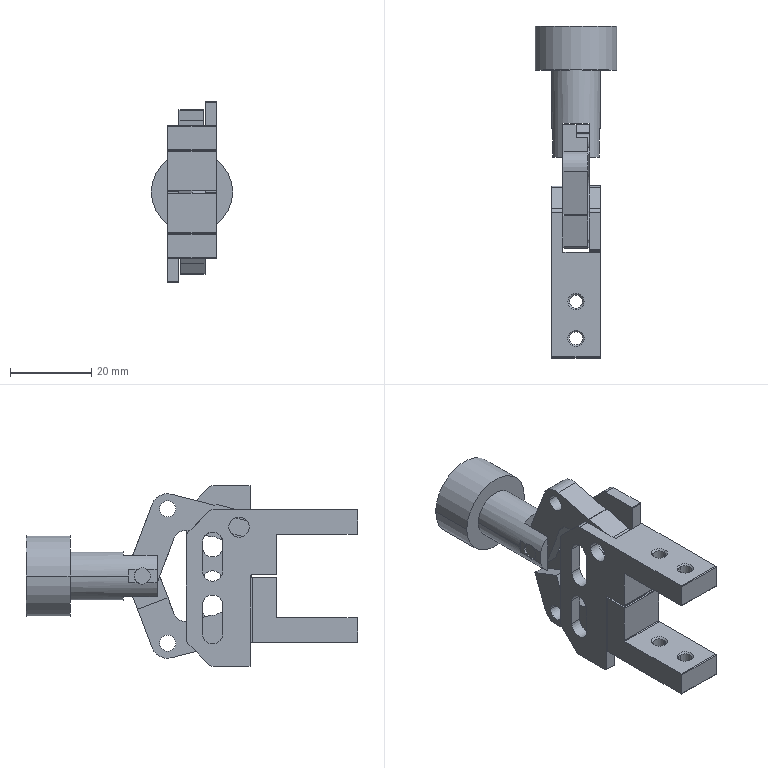Component | SolidWorks | CCDJSHFP20(NC)+(CS1-G-2)-1_CCDJSHFP20_finger(0)-1 | 1 solid | 194 faces | box 20 x 81.5 x 44.3 mm | volume 15573 mm3 | plane 107 | cylinder 71 | cone 16 | commonest cylinder face diameters 4 x16 5 x12 0.4 x12 3.242 x8 3 x8 1 x5 4.2 x2 20 x2
build123d program:
from build123d import *

# Parameters (mm, degrees)
CUT_EXTRUDE1_2_DEPTH      = 6
CUT_EXTRUDE1_2_DEPTH_BACK = 6
CUT_EXTRUDE2_DEPTH        = 6
CUT_EXTRUDE2_DEPTH_BACK   = 6
SKETCH3_R                 = 2
SKETCH4_R                 = 2
BOSS_EXTRUDE1_DEPTH       = 3.2
SKETCH5_R                 = 2
BOSS_EXTRUDE2_DEPTH       = 6.1
SKETCH6_R                 = 2
BOSS_EXTRUDE3_DEPTH       = 3.2
SKETCH7_R                 = 2
BOSS_EXTRUDE4_DEPTH       = 6.1
SKETCH8_R                 = 2.5
BOSS_EXTRUDE5_DEPTH       = 2.8
BOSS_EXTRUDE6_START       = 11.7
BOSS_EXTRUDE6_DEPTH       = 11.7
SKETCH10_R                = 2.5
BOSS_EXTRUDE7_DEPTH       = 2.8
BOSS_EXTRUDE8_DEPTH       = 12
BOSS_EXTRUDE9_DEPTH       = 5.35
BOSS_EXTRUDE9_DEPTH_BACK  = 5.35
SKETCH12_R                = 2.1
CUT_EXTRUDE1_DEPTH        = 66.663
CUT_EXTRUDE1_DEPTH_BACK   = 66.663
SKETCH1_R                 = 2


with BuildPart() as part:
    # Sketch1_2 → Revolve1 (revolve)
    with BuildSketch(Plane.XY, mode=Mode.PRIVATE) as revolve1_sk:
        Polygon((28.8, 0), (28.8, 6), (50.2, 6), (50.2, 10), (61, 10), (61, 0), align=None)
    revolve(revolve1_sk.sketch.rotate(Axis((61, 0, 0), (-1, 0, 0)), 270), axis=Axis((61, 0, 0), (-1, 0, 0)))

    # Sketch2 → Cut-Extrude1_2 (cut, two sides: drawn at the far end of the back side and taken through both)
    with BuildSketch(Plane(origin=(0, 0, 0), x_dir=(1, 0, 0), z_dir=(0, 1, 0)).offset(-CUT_EXTRUDE1_2_DEPTH_BACK)):
        Polygon((26.8, -6), (35.8, -6), (35.8, -5.75), (28.8, -5.75), (28.8, -3.2), (37.1, -3.2), (37.1, 3.2), (28.8, 3.2), (28.8, 5.75), (35.8, 5.75), (35.8, 6), (26.8, 6), align=None)
    extrude(amount=CUT_EXTRUDE1_2_DEPTH + CUT_EXTRUDE1_2_DEPTH_BACK, mode=Mode.SUBTRACT)

    # Sketch3 → Cut-Extrude2 (cut, two sides: drawn at the far end of the back side and taken through both)
    with BuildSketch(Plane.XY.offset(-CUT_EXTRUDE2_DEPTH_BACK)):
        with Locations(Location((32.45, 0, 0), (0, 0, 58.977))):
            Circle(SKETCH3_R)
    extrude(amount=CUT_EXTRUDE2_DEPTH + CUT_EXTRUDE2_DEPTH_BACK, mode=Mode.SUBTRACT)

    # Sketch4 → Boss-Extrude1 (add)
    with BuildSketch(Plane.XY.offset(-3.2)):
        with BuildLine():
            Line((20.984, 18.979), (29.329, -3.053))
            Line((29.329, -3.053), (31.2, -2.345))
            Line((31.2, -2.345), (29.96, 0.9281))
            ThreePointArc((29.96, 0.9281), (31.122, 3.507), (33.7, 2.345))
            Line((33.7, 2.345), (34.94, -0.9281))
            Line((34.94, -0.9281), (36.811, -0.2196))
            Line((36.811, -0.2196), (30.048, 17.635))
            ThreePointArc((30.048, 17.635), (28.149, 19.768), (25.311, 20.092))
            Line((25.311, 20.092), (20.984, 18.979))
        make_face()
        with Locations((26.2, 16.5)):
            Circle(SKETCH4_R, mode=Mode.SUBTRACT)
    extrude(amount=BOSS_EXTRUDE1_DEPTH)

    # Sketch5 → Boss-Extrude2 (add)
    with BuildSketch(Plane.XY.offset(-3.2)):
        with BuildLine():
            Line((6.434, 15.031), (6.807, 13.578))
            Line((6.807, 13.578), (9.229, 14.201))
            ThreePointArc((9.229, 14.201), (11.664, 12.762), (10.225, 10.327))
            Line((10.225, 10.327), (7.803, 9.704))
            Line((7.803, 9.704), (8.177, 8.252))
            ThreePointArc((8.177, 8.252), (8.407, 7.946), (8.786, 7.892))
            Line((8.786, 7.892), (21.127, 11.065))
            ThreePointArc((21.127, 11.065), (23.255, 10.823), (24.679, 9.223))
            Line((24.679, 9.223), (26.141, 5.363))
            Line((26.141, 5.363), (33.622, 8.197))
            Line((33.622, 8.197), (30.048, 17.635))
            ThreePointArc((30.048, 17.635), (28.149, 19.768), (25.311, 20.092))
            Line((25.311, 20.092), (14.713, 17.367))
            Line((14.713, 17.367), (14.348, 17.582))
            Line((14.348, 17.582), (6.793, 15.64))
            ThreePointArc((6.793, 15.64), (6.488, 15.41), (6.434, 15.031))
        make_face()
        with Locations((26.2, 16.5)):
            Circle(SKETCH5_R, mode=Mode.SUBTRACT)
    extrude(amount=BOSS_EXTRUDE2_DEPTH)

    # Sketch6 → Boss-Extrude3 (add)
    with BuildSketch(Plane.XY.offset(3.2)):
        with BuildLine():
            Line((20.984, -18.979), (25.311, -20.092))
            ThreePointArc((25.311, -20.092), (28.149, -19.768), (30.048, -17.635))
            Line((30.048, -17.635), (36.811, 0.2196))
            Line((36.811, 0.2196), (34.94, 0.9281))
            Line((34.94, 0.9281), (33.7, -2.345))
            ThreePointArc((33.7, -2.345), (31.122, -3.507), (29.96, -0.9281))
            Line((29.96, -0.9281), (31.2, 2.345))
            Line((31.2, 2.345), (29.329, 3.053))
            Line((29.329, 3.053), (20.984, -18.979))
        make_face()
        with Locations((26.2, -16.5)):
            Circle(SKETCH6_R, mode=Mode.SUBTRACT)
    extrude(amount=-BOSS_EXTRUDE3_DEPTH)

    # Sketch7 → Boss-Extrude4 (add)
    with BuildSketch(Plane.XY.offset(3.2)):
        with BuildLine():
            Line((6.793, -15.64), (14.348, -17.582))
            Line((14.348, -17.582), (14.713, -17.367))
            Line((14.713, -17.367), (25.311, -20.092))
            ThreePointArc((25.311, -20.092), (28.149, -19.768), (30.048, -17.635))
            Line((30.048, -17.635), (33.622, -8.197))
            Line((33.622, -8.197), (26.141, -5.363))
            Line((26.141, -5.363), (24.679, -9.223))
            ThreePointArc((24.679, -9.223), (23.255, -10.823), (21.127, -11.065))
            Line((21.127, -11.065), (8.786, -7.892))
            ThreePointArc((8.786, -7.892), (8.407, -7.946), (8.177, -8.252))
            Line((8.177, -8.252), (7.803, -9.704))
            Line((7.803, -9.704), (10.225, -10.327))
            ThreePointArc((10.225, -10.327), (11.664, -12.762), (9.229, -14.201))
            Line((9.229, -14.201), (6.807, -13.578))
            Line((6.807, -13.578), (6.434, -15.031))
            ThreePointArc((6.434, -15.031), (6.488, -15.41), (6.793, -15.64))
        make_face()
        with Locations((26.2, -16.5)):
            Circle(SKETCH7_R, mode=Mode.SUBTRACT)
    extrude(amount=-BOSS_EXTRUDE4_DEPTH)

    # Sketch8 → Boss-Extrude5 (add)
    with BuildSketch(Plane.XY.offset(-3.2)):
        with BuildLine():
            Line((-20.5, 16.05), (-20.5, 10.45))
            ThreePointArc((-20.5, 10.45), (-20.441, 10.309), (-20.3, 10.25))
            Line((-20.3, 10.25), (-0.7, 10.25))
            ThreePointArc((-0.7, 10.25), (-0.5586, 10.191), (-0.5, 10.05))
            Line((-0.5, 10.05), (-0.5, 0.45))
            ThreePointArc((-0.5, 0.45), (-0.4414, 0.3086), (-0.3, 0.25))
            Line((-0.3, 0.25), (5.6, 0.25))
            ThreePointArc((5.6, 0.25), (5.741, 0.1914), (5.8, 0.05))
            Line((5.8, 0.05), (5.8, -21.95))
            ThreePointArc((5.8, -21.95), (5.859, -22.091), (6, -22.15))
            Line((6, -22.15), (15.079, -22.15))
            ThreePointArc((15.079, -22.15), (15.653, -22.036), (16.139, -21.711))
            Line((16.139, -21.711), (21.261, -16.589))
            ThreePointArc((21.261, -16.589), (21.586, -16.103), (21.7, -15.529))
            Line((21.7, -15.529), (21.7, 9.629))
            ThreePointArc((21.7, 9.629), (21.586, 10.203), (21.261, 10.689))
            Line((21.261, 10.689), (16.139, 15.811))
            ThreePointArc((16.139, 15.811), (15.653, 16.136), (15.079, 16.25))
            Line((15.079, 16.25), (-20.3, 16.25))
            ThreePointArc((-20.3, 16.25), (-20.441, 16.191), (-20.5, 16.05))
        make_face()
        with Locations((8.7, 12)):
            Circle(SKETCH8_R, mode=Mode.SUBTRACT)
        with BuildLine():
            Line((12.7, -7.15), (12.7, -14.15))
            ThreePointArc((12.7, -14.15), (15.2, -16.65), (17.7, -14.15))
            Line((17.7, -14.15), (17.7, -7.15))
            ThreePointArc((17.7, -7.15), (15.2, -4.65), (12.7, -7.15))
        make_face(mode=Mode.SUBTRACT)
        with BuildLine():
            Line((12.7, 8.25), (12.7, 1.25))
            ThreePointArc((12.7, 1.25), (15.2, -1.25), (17.7, 1.25))
            Line((17.7, 1.25), (17.7, 8.25))
            ThreePointArc((17.7, 8.25), (15.2, 10.75), (12.7, 8.25))
        make_face(mode=Mode.SUBTRACT)
    extrude(amount=-BOSS_EXTRUDE5_DEPTH)

    # Sketch9 → Boss-Extrude6 (add)
    with BuildSketch(Plane.XY.offset(-5.7).offset(BOSS_EXTRUDE6_START)):
        with BuildLine():
            Line((-20.5, 16.05), (-20.5, 10.45))
            ThreePointArc((-20.5, 10.45), (-20.441, 10.309), (-20.3, 10.25))
            Line((-20.3, 10.25), (-0.7, 10.25))
            ThreePointArc((-0.7, 10.25), (-0.5586, 10.191), (-0.5, 10.05))
            Line((-0.5, 10.05), (-0.5, 0.45))
            ThreePointArc((-0.5, 0.45), (-0.4414, 0.3086), (-0.3, 0.25))
            Line((-0.3, 0.25), (5.4, 0.25))
            Line((5.4, 0.25), (5.4, 16.25))
            Line((5.4, 16.25), (-20.3, 16.25))
            ThreePointArc((-20.3, 16.25), (-20.441, 16.191), (-20.5, 16.05))
        make_face()
    extrude(amount=-BOSS_EXTRUDE6_DEPTH)

    # Sketch10 → Boss-Extrude7 (add)
    with BuildSketch(Plane.XY.offset(3.2)):
        with BuildLine():
            Line((-20.3, -16.25), (15.079, -16.25))
            ThreePointArc((15.079, -16.25), (15.653, -16.136), (16.139, -15.811))
            Line((16.139, -15.811), (21.261, -10.689))
            ThreePointArc((21.261, -10.689), (21.586, -10.203), (21.7, -9.629))
            Line((21.7, -9.629), (21.7, 15.529))
            ThreePointArc((21.7, 15.529), (21.586, 16.103), (21.261, 16.589))
            Line((21.261, 16.589), (16.139, 21.711))
            ThreePointArc((16.139, 21.711), (15.653, 22.036), (15.079, 22.15))
            Line((15.079, 22.15), (6, 22.15))
            ThreePointArc((6, 22.15), (5.859, 22.091), (5.8, 21.95))
            Line((5.8, 21.95), (5.8, -0.05))
            ThreePointArc((5.8, -0.05), (5.741, -0.1914), (5.6, -0.25))
            Line((5.6, -0.25), (-0.3, -0.25))
            ThreePointArc((-0.3, -0.25), (-0.4414, -0.3086), (-0.5, -0.45))
            Line((-0.5, -0.45), (-0.5, -10.05))
            ThreePointArc((-0.5, -10.05), (-0.5586, -10.191), (-0.7, -10.25))
            Line((-0.7, -10.25), (-20.3, -10.25))
            ThreePointArc((-20.3, -10.25), (-20.441, -10.309), (-20.5, -10.45))
            Line((-20.5, -10.45), (-20.5, -16.05))
            ThreePointArc((-20.5, -16.05), (-20.441, -16.191), (-20.3, -16.25))
        make_face()
        with Locations(Location((8.7, -12, 0), (0, 0, 220.41))):
            Circle(SKETCH10_R, mode=Mode.SUBTRACT)
        with BuildLine():
            Line((17.7, 7.15), (17.7, 14.15))
            ThreePointArc((17.7, 14.15), (15.2, 16.65), (12.7, 14.15))
            Line((12.7, 14.15), (12.7, 7.15))
            ThreePointArc((12.7, 7.15), (15.2, 4.65), (17.7, 7.15))
        make_face(mode=Mode.SUBTRACT)
        with BuildLine():
            Line((17.7, -8.25), (17.7, -1.25))
            ThreePointArc((17.7, -1.25), (15.2, 1.25), (12.7, -1.25))
            Line((12.7, -1.25), (12.7, -8.25))
            ThreePointArc((12.7, -8.25), (15.2, -10.75), (17.7, -8.25))
        make_face(mode=Mode.SUBTRACT)
    extrude(amount=BOSS_EXTRUDE7_DEPTH)

    # Sketch11 → Boss-Extrude8 (add)
    with BuildSketch(Plane.XY.offset(-6)):
        with BuildLine():
            Line((-20.3, -16.25), (5.4, -16.25))
            Line((5.4, -16.25), (5.4, -0.25))
            Line((5.4, -0.25), (-0.3, -0.25))
            ThreePointArc((-0.3, -0.25), (-0.4414, -0.3086), (-0.5, -0.45))
            Line((-0.5, -0.45), (-0.5, -10.05))
            ThreePointArc((-0.5, -10.05), (-0.5586, -10.191), (-0.7, -10.25))
            Line((-0.7, -10.25), (-20.3, -10.25))
            ThreePointArc((-20.3, -10.25), (-20.441, -10.309), (-20.5, -10.45))
            Line((-20.5, -10.45), (-20.5, -16.05))
            ThreePointArc((-20.5, -16.05), (-20.441, -16.191), (-20.3, -16.25))
        make_face()
    extrude(amount=BOSS_EXTRUDE8_DEPTH)

    # Sketch12 → Boss-Extrude9 (add, two sides: drawn at the far end of the back side and taken through both)
    with BuildSketch(Plane.XY.offset(-BOSS_EXTRUDE9_DEPTH_BACK)):
        with Locations(Location((32.45, 0, 0), (0, 0, 182.993))):
            Circle(SKETCH12_R)
    extrude(amount=BOSS_EXTRUDE9_DEPTH + BOSS_EXTRUDE9_DEPTH_BACK)

    # Sketch13 → Cut-Revolve1 (revolve, cut)
    with BuildSketch(Plane.XY, mode=Mode.PRIVATE) as cut_revolve1_sk:
        Polygon((-15.7, 16.25), (-13.7, 16.25), (-14.079, 15.871), (-14.079, 10.629), (-13.7, 10.25), (-15.7, 10.25), align=None)
    revolve(cut_revolve1_sk.sketch.rotate(Axis((-15.7, 10.25, 0), (0, 1, 0)), 180), axis=Axis((-15.7, 10.25, 0), (0, 1, 0)), mode=Mode.SUBTRACT)

    # Sketch14 → Cut-Revolve2 (revolve, cut)
    with BuildSketch(Plane.XY, mode=Mode.PRIVATE) as cut_revolve2_sk:
        Polygon((-6.7, 16.25), (-4.7, 16.25), (-5.079, 15.871), (-5.079, 10.629), (-4.7, 10.25), (-6.7, 10.25), align=None)
    revolve(cut_revolve2_sk.sketch.rotate(Axis((-6.7, 10.25, 0), (0, 1, 0)), 270), axis=Axis((-6.7, 10.25, 0), (0, 1, 0)), mode=Mode.SUBTRACT)

    # Sketch15 → Cut-Revolve3 (revolve, cut)
    with BuildSketch(Plane.XY, mode=Mode.PRIVATE) as cut_revolve3_sk:
        Polygon((-15.7, -10.25), (-13.7, -10.25), (-14.079, -10.629), (-14.079, -15.871), (-13.7, -16.25), (-15.7, -16.25), align=None)
    revolve(cut_revolve3_sk.sketch.rotate(Axis((-15.7, -16.25, 0), (0, 1, 0)), 180), axis=Axis((-15.7, -16.25, 0), (0, 1, 0)), mode=Mode.SUBTRACT)

    # Sketch16 → Cut-Revolve4 (revolve, cut)
    with BuildSketch(Plane.XY, mode=Mode.PRIVATE) as cut_revolve4_sk:
        Polygon((-6.7, -10.25), (-4.7, -10.25), (-5.079, -10.629), (-5.079, -15.871), (-4.7, -16.25), (-6.7, -16.25), align=None)
    revolve(cut_revolve4_sk.sketch.rotate(Axis((-6.7, -16.25, 0), (0, 1, 0)), 270), axis=Axis((-6.7, -16.25, 0), (0, 1, 0)), mode=Mode.SUBTRACT)

    # Sketch1 → Cut-Extrude1 (cut, two sides: drawn at the far end of the back side and taken through both)
    with BuildSketch(Plane.XY.offset(-CUT_EXTRUDE1_DEPTH_BACK)):
        with Locations((15.2, 7.7)):
            Circle(SKETCH1_R)
        with Locations((15.2, -7.7)):
            Circle(SKETCH1_R)
    extrude(amount=CUT_EXTRUDE1_DEPTH + CUT_EXTRUDE1_DEPTH_BACK, mode=Mode.SUBTRACT)


solid = part.part

# Placed as in the assembly
solid = solid.moved(Location((-158.9, 291.364, -122.57), (90, 90, 0)))